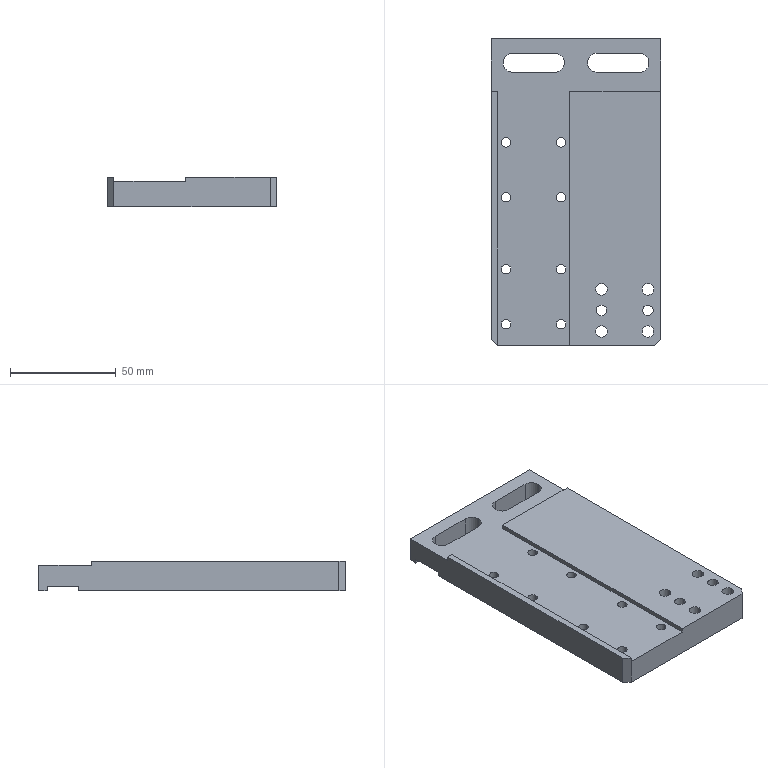Component | SolidWorks | H2020022-0418-1-1 | 1 solid | 100 faces | box 80 x 145 x 14 mm | volume 136861 mm3 | cylinder 62 | plane 34 | cone 4 | commonest cylinder face diameters 8 x16 4.5 x16 10 x8 5.5 x8 9 x6 3.3 x4 5 x4 | material 6061 Aluminum Alloy
build123d program:
from build123d import *

# Parameters (mm, degrees)
SKETCH1_W                                       = 80
SKETCH1_H                                       = 145
BOSS_EXTRUDE1_DEPTH                             = 14
SKETCH2_W                                       = 34
SKETCH2_H                                       = 145
CUT_EXTRUDE1_DEPTH                              = 2
M4_HEX_SOCKET_HEAD_CAP_SCREW_CBORE1_D           = 4.5
M4_HEX_SOCKET_HEAD_CAP_SCREW_CBORE1_CBORE_D     = 8
M4_HEX_SOCKET_HEAD_CAP_SCREW_CBORE1_CBORE_DEPTH = 4.4
CHAMFER1_SIZE                                   = 3
M5_HEX_SOCKET_HEAD_CAP_SCREW_CBORE1_D           = 5.5
M5_HEX_SOCKET_HEAD_CAP_SCREW_CBORE1_CBORE_D     = 10
M5_HEX_SOCKET_HEAD_CAP_SCREW_CBORE1_CBORE_DEPTH = 5.4
SKETCH12_R                                      = 2.5
CUT_EXTRUDE3_DEPTH                              = 167.196
M4_TAPPED_HOLE1_D                               = 3.3
M4_TAPPED_HOLE1_DEPTH                           = 12.1
M4_TAPPED_HOLE1_TIP                             = 0.9914
SKETCH15_W                                      = 80
SKETCH15_H                                      = 14.8
CUT_EXTRUDE4_DEPTH                              = 2
LPATTERN1_COUNT                                 = 2
LPATTERN1_PITCH                                 = 60
CUT_EXTRUDE5_DEPTH                              = 167.196
SKETCH17_W                                      = 80
SKETCH17_H                                      = 25
CUT_EXTRUDE6_DEPTH                              = 2


with BuildPart() as part:
    # Sketch1 → Boss-Extrude1 (new body)
    with BuildSketch(Plane(origin=(0, 0, 0), x_dir=(0, 0, -1), z_dir=(1, 0, 0))):
        with Locations((40, -72.5)):
            Rectangle(SKETCH1_W, SKETCH1_H)
    extrude(amount=BOSS_EXTRUDE1_DEPTH)

    # Sketch2 → Cut-Extrude1 (cut)
    with BuildSketch(Plane(origin=(14, 0, 0), x_dir=(0, 0, -1), z_dir=(1, 0, 0))):
        with Locations((20, -72.5)):
            Rectangle(SKETCH2_W, SKETCH2_H)
    extrude(amount=-CUT_EXTRUDE1_DEPTH, mode=Mode.SUBTRACT)

    # M4 Hex Socket Head Cap Screw CBORE1 (through all)
    with Locations(Plane.ZY):
        with Locations((-33, -109), (-7, -109), (-7, -135), (-33, -135)):
            m4_hex_socket_head_cap_screw_cbore1 = CounterBoreHole(M4_HEX_SOCKET_HEAD_CAP_SCREW_CBORE1_D / 2, M4_HEX_SOCKET_HEAD_CAP_SCREW_CBORE1_CBORE_D / 2, M4_HEX_SOCKET_HEAD_CAP_SCREW_CBORE1_CBORE_DEPTH)

    # Chamfer1
    chamfer1_edges = [part.edges().sort_by_distance(p)[0] for p in [
        (7, -145, -80),
        (7, -145, 0),
    ]]
    chamfer(chamfer1_edges, length=CHAMFER1_SIZE)

    # M5 Hex Socket Head Cap Screw CBORE1 (through all)
    with Locations(Plane.ZY):
        with Locations((-74, -138.5), (-52, -138.5), (-52, -118.5), (-74, -118.5)):
            CounterBoreHole(M5_HEX_SOCKET_HEAD_CAP_SCREW_CBORE1_D / 2, M5_HEX_SOCKET_HEAD_CAP_SCREW_CBORE1_CBORE_D / 2, M5_HEX_SOCKET_HEAD_CAP_SCREW_CBORE1_CBORE_DEPTH)

    # Sketch12 → Cut-Extrude3 (cut, through all)
    with BuildSketch(Plane.ZY):
        with Locations((-74, -128.5)):
            Circle(SKETCH12_R)
        with Locations((-52, -128.5)):
            Circle(SKETCH12_R)
    extrude(amount=-CUT_EXTRUDE3_DEPTH, mode=Mode.SUBTRACT)

    # M4 Tapped Hole1
    with Locations(Plane(origin=(0, 0, -80), x_dir=(-1, 0, 0), z_dir=(0, 0, -1))):
        with Locations((-7, -35), (-7, -55)):
            Hole(M4_TAPPED_HOLE1_D / 2, depth=M4_TAPPED_HOLE1_DEPTH)
            with Locations((0, 0, -(M4_TAPPED_HOLE1_DEPTH + M4_TAPPED_HOLE1_TIP / 2))):  # 118° drill point
                Cone(0, M4_TAPPED_HOLE1_D / 2, M4_TAPPED_HOLE1_TIP, mode=Mode.SUBTRACT)

    # Sketch15 → Cut-Extrude4 (cut)
    with BuildSketch(Plane.ZY):
        with Locations((-40, -11.4)):
            Rectangle(SKETCH15_W, SKETCH15_H)
    extrude(amount=-CUT_EXTRUDE4_DEPTH, mode=Mode.SUBTRACT)

    # LPattern1: M4 Hex Socket Head Cap Screw CBORE1 ×2
    with Locations(*[(0, i * LPATTERN1_PITCH, 0) for i in range(1, LPATTERN1_COUNT)]):
        add(m4_hex_socket_head_cap_screw_cbore1, mode=Mode.SUBTRACT)

    # Sketch16 → Cut-Extrude5 (cut, through all)
    with BuildSketch(Plane(origin=(14, 0, 0), x_dir=(0, 0, -1), z_dir=(1, 0, 0))):
        with BuildLine():
            Line((50, -6.9), (70, -6.9))
            ThreePointArc((70, -6.9), (74.5, -11.4), (70, -15.9))
            Line((70, -15.9), (50, -15.9))
            ThreePointArc((50, -15.9), (45.5, -11.4), (50, -6.9))
        make_face()
        with BuildLine():
            Line((10, -6.9), (30, -6.9))
            ThreePointArc((30, -6.9), (34.5, -11.4), (30, -15.9))
            Line((30, -15.9), (10, -15.9))
            ThreePointArc((10, -15.9), (5.5, -11.4), (10, -6.9))
        make_face()
    extrude(amount=-CUT_EXTRUDE5_DEPTH, mode=Mode.SUBTRACT)

    # Sketch17 → Cut-Extrude6 (cut)
    with BuildSketch(Plane(origin=(14, 0, 0), x_dir=(0, 0, -1), z_dir=(1, 0, 0))):
        with Locations((40, -12.5)):
            Rectangle(SKETCH17_W, SKETCH17_H)
    extrude(amount=-CUT_EXTRUDE6_DEPTH, mode=Mode.SUBTRACT)


solid = part.part

# Placed as in the assembly
solid = solid.moved(Location((-68.068, 120.813, 376.197), (0, -90, 0)))